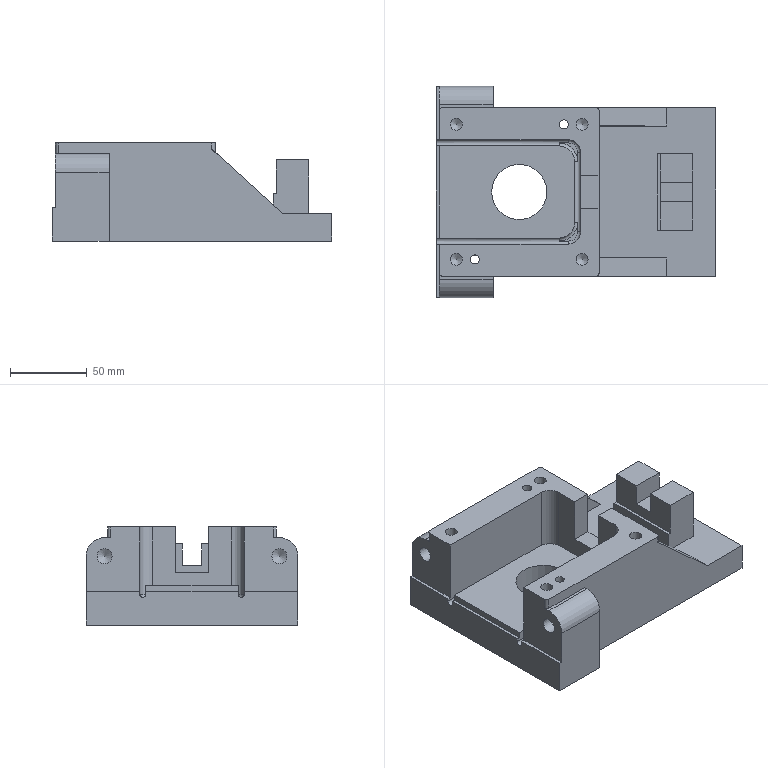Component | NX | FIXTURE_BODY | 1 solid | 80 faces | volume 708418 mm3 | plane 48 | cylinder 22 | cone 6 | torus 4 | commonest cylinder face diameters 4 x7 7.8 x4 24 x2 16 x2 20 x2 6 x2 9.8 x2 36 x1